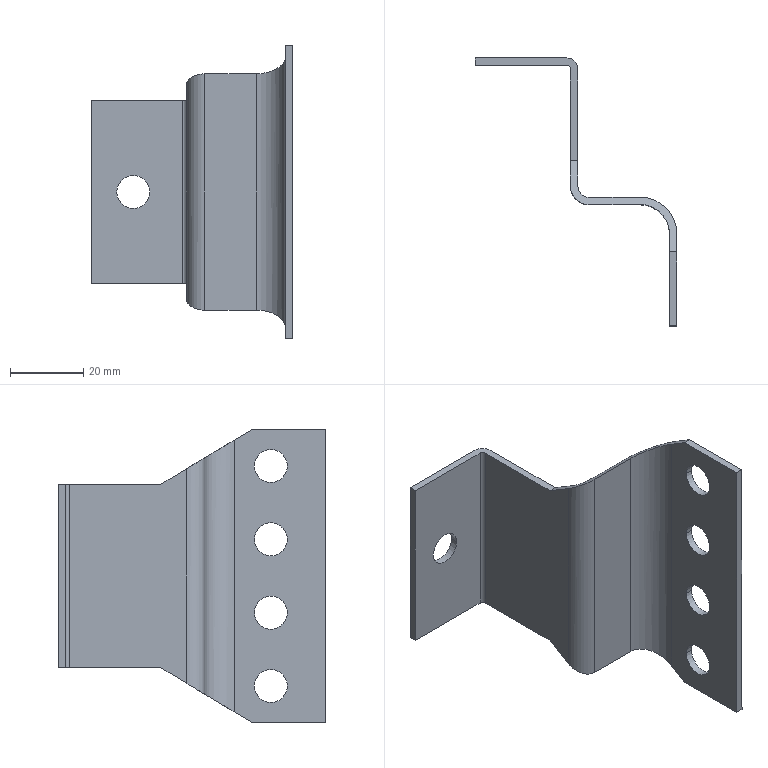Component | SolidWorks | 500CabinetWidthDoorCrossbeamAssembly-1_Connector-1 | 1 solid | 32 faces | box 55 x 73 x 80 mm | volume 13851 mm3 | cylinder 16 | plane 16 | commonest cylinder face diameters 9 x10 6 x2 20 x1 16 x1 10 x1 2 x1 | material Plain Carbon Steel
STEP:
#1=COLOUR_RGB('',0.7922,0.8196,0.9333);
#2=FILL_AREA_STYLE_COLOUR('',#1);
#3=FILL_AREA_STYLE('',(#2));
#4=SURFACE_STYLE_FILL_AREA(#3);
#5=SURFACE_SIDE_STYLE('',(#4));
#6=SURFACE_STYLE_USAGE(.BOTH.,#5);
#7=PRESENTATION_STYLE_ASSIGNMENT((#6));
#8=CARTESIAN_POINT('',(-49.801,4.761,85.05));
#9=VERTEX_POINT('',#8);
#10=CARTESIAN_POINT('',(-49.801,4.406,85.05));
#11=VERTEX_POINT('',#10);
#12=CARTESIAN_POINT('',(-49.801,4.583,85.05));
#13=DIRECTION('',(1.,0.,0.));
#14=DIRECTION('',(0.,-1.,0.));
#15=AXIS2_PLACEMENT_3D('',#12,#13,#14);
#16=CIRCLE('',#15,0.1772);
#17=EDGE_CURVE('',#9,#11,#16,.T.);
#18=ORIENTED_EDGE('',*,*,#17,.F.);
#19=CARTESIAN_POINT('',(-49.722,4.761,85.05));
#20=VERTEX_POINT('',#19);
#21=CARTESIAN_POINT('',(-52.872,4.761,85.05));
#22=DIRECTION('',(1.,-0.,0.));
#23=VECTOR('',#22,39.37);
#24=LINE('',#21,#23);
#25=EDGE_CURVE('',#9,#20,#24,.T.);
#26=ORIENTED_EDGE('',*,*,#25,.T.);
#27=CARTESIAN_POINT('',(-49.722,4.406,85.05));
#28=VERTEX_POINT('',#27);
#29=CARTESIAN_POINT('',(-49.722,4.583,85.05));
#30=DIRECTION('',(1.,-0.,0.));
#31=DIRECTION('',(0.,-1.,0.));
#32=AXIS2_PLACEMENT_3D('',#29,#30,#31);
#33=CIRCLE('',#32,0.1772);
#34=EDGE_CURVE('',#20,#28,#33,.T.);
#35=ORIENTED_EDGE('',*,*,#34,.T.);
#36=CARTESIAN_POINT('',(-52.872,4.406,85.05));
#37=DIRECTION('',(1.,-0.,0.));
#38=VECTOR('',#37,39.37);
#39=LINE('',#36,#38);
#40=EDGE_CURVE('',#11,#28,#39,.T.);
#41=ORIENTED_EDGE('',*,*,#40,.F.);
#42=EDGE_LOOP('',(#18,#26,#35,#41));
#43=FACE_OUTER_BOUND('',#42,.T.);
#44=CARTESIAN_POINT('',(-52.872,4.583,85.05));
#45=DIRECTION('',(1.,-0.,0.));
#46=DIRECTION('',(0.,-1.,0.));
#47=AXIS2_PLACEMENT_3D('',#44,#45,#46);
#48=CYLINDRICAL_SURFACE('',#47,0.1772);
#49=ADVANCED_FACE('',(#43),#48,.F.);
#50=CARTESIAN_POINT('',(-49.801,4.761,87.412));
#51=VERTEX_POINT('',#50);
#52=CARTESIAN_POINT('',(-49.801,4.406,87.412));
#53=VERTEX_POINT('',#52);
#54=CARTESIAN_POINT('',(-49.801,4.583,87.412));
#55=DIRECTION('',(1.,0.,0.));
#56=DIRECTION('',(0.,-1.,0.));
#57=AXIS2_PLACEMENT_3D('',#54,#55,#56);
#58=CIRCLE('',#57,0.1772);
#59=EDGE_CURVE('',#51,#53,#58,.T.);
#60=ORIENTED_EDGE('',*,*,#59,.F.);
#61=CARTESIAN_POINT('',(-49.722,4.761,87.412));
#62=VERTEX_POINT('',#61);
#63=CARTESIAN_POINT('',(-52.872,4.761,87.412));
#64=DIRECTION('',(1.,-0.,0.));
#65=VECTOR('',#64,39.37);
#66=LINE('',#63,#65);
#67=EDGE_CURVE('',#51,#62,#66,.T.);
#68=ORIENTED_EDGE('',*,*,#67,.T.);
#69=CARTESIAN_POINT('',(-49.722,4.406,87.412));
#70=VERTEX_POINT('',#69);
#71=CARTESIAN_POINT('',(-49.722,4.583,87.412));
#72=DIRECTION('',(1.,-0.,0.));
#73=DIRECTION('',(0.,-1.,0.));
#74=AXIS2_PLACEMENT_3D('',#71,#72,#73);
#75=CIRCLE('',#74,0.1772);
#76=EDGE_CURVE('',#62,#70,#75,.T.);
#77=ORIENTED_EDGE('',*,*,#76,.T.);
#78=CARTESIAN_POINT('',(-52.872,4.406,87.412));
#79=DIRECTION('',(1.,-0.,0.));
#80=VECTOR('',#79,39.37);
#81=LINE('',#78,#80);
#82=EDGE_CURVE('',#53,#70,#81,.T.);
#83=ORIENTED_EDGE('',*,*,#82,.F.);
#84=EDGE_LOOP('',(#60,#68,#77,#83));
#85=FACE_OUTER_BOUND('',#84,.T.);
#86=CARTESIAN_POINT('',(-52.872,4.583,87.412));
#87=DIRECTION('',(1.,-0.,0.));
#88=DIRECTION('',(0.,-1.,0.));
#89=AXIS2_PLACEMENT_3D('',#86,#87,#88);
#90=CYLINDRICAL_SURFACE('',#89,0.1772);
#91=ADVANCED_FACE('',(#85),#90,.F.);
#92=CARTESIAN_POINT('',(-49.801,4.761,86.625));
#93=VERTEX_POINT('',#92);
#94=CARTESIAN_POINT('',(-49.801,4.406,86.625));
#95=VERTEX_POINT('',#94);
#96=CARTESIAN_POINT('',(-49.801,4.583,86.625));
#97=DIRECTION('',(1.,0.,0.));
#98=DIRECTION('',(0.,-1.,0.));
#99=AXIS2_PLACEMENT_3D('',#96,#97,#98);
#100=CIRCLE('',#99,0.1772);
#101=EDGE_CURVE('',#93,#95,#100,.T.);
#102=ORIENTED_EDGE('',*,*,#101,.F.);
#103=CARTESIAN_POINT('',(-49.722,4.761,86.625));
#104=VERTEX_POINT('',#103);
#105=CARTESIAN_POINT('',(-52.872,4.761,86.625));
#106=DIRECTION('',(1.,-0.,0.));
#107=VECTOR('',#106,39.37);
#108=LINE('',#105,#107);
#109=EDGE_CURVE('',#93,#104,#108,.T.);
#110=ORIENTED_EDGE('',*,*,#109,.T.);
#111=CARTESIAN_POINT('',(-49.722,4.406,86.625));
#112=VERTEX_POINT('',#111);
#113=CARTESIAN_POINT('',(-49.722,4.583,86.625));
#114=DIRECTION('',(1.,-0.,0.));
#115=DIRECTION('',(0.,-1.,0.));
#116=AXIS2_PLACEMENT_3D('',#113,#114,#115);
#117=CIRCLE('',#116,0.1772);
#118=EDGE_CURVE('',#104,#112,#117,.T.);
#119=ORIENTED_EDGE('',*,*,#118,.T.);
#120=CARTESIAN_POINT('',(-52.872,4.406,86.625));
#121=DIRECTION('',(1.,-0.,0.));
#122=VECTOR('',#121,39.37);
#123=LINE('',#120,#122);
#124=EDGE_CURVE('',#95,#112,#123,.T.);
#125=ORIENTED_EDGE('',*,*,#124,.F.);
#126=EDGE_LOOP('',(#102,#110,#119,#125));
#127=FACE_OUTER_BOUND('',#126,.T.);
#128=CARTESIAN_POINT('',(-52.872,4.583,86.625));
#129=DIRECTION('',(1.,-0.,0.));
#130=DIRECTION('',(0.,-1.,0.));
#131=AXIS2_PLACEMENT_3D('',#128,#129,#130);
#132=CYLINDRICAL_SURFACE('',#131,0.1772);
#133=ADVANCED_FACE('',(#127),#132,.F.);
#134=CARTESIAN_POINT('',(-49.801,4.761,85.837));
#135=VERTEX_POINT('',#134);
#136=CARTESIAN_POINT('',(-49.801,4.406,85.837));
#137=VERTEX_POINT('',#136);
#138=CARTESIAN_POINT('',(-49.801,4.583,85.837));
#139=DIRECTION('',(1.,0.,0.));
#140=DIRECTION('',(0.,-1.,0.));
#141=AXIS2_PLACEMENT_3D('',#138,#139,#140);
#142=CIRCLE('',#141,0.1772);
#143=EDGE_CURVE('',#135,#137,#142,.T.);
#144=ORIENTED_EDGE('',*,*,#143,.F.);
#145=CARTESIAN_POINT('',(-49.722,4.761,85.837));
#146=VERTEX_POINT('',#145);
#147=CARTESIAN_POINT('',(-52.872,4.761,85.837));
#148=DIRECTION('',(1.,-0.,0.));
#149=VECTOR('',#148,39.37);
#150=LINE('',#147,#149);
#151=EDGE_CURVE('',#135,#146,#150,.T.);
#152=ORIENTED_EDGE('',*,*,#151,.T.);
#153=CARTESIAN_POINT('',(-49.722,4.406,85.837));
#154=VERTEX_POINT('',#153);
#155=CARTESIAN_POINT('',(-49.722,4.583,85.837));
#156=DIRECTION('',(1.,-0.,0.));
#157=DIRECTION('',(0.,-1.,0.));
#158=AXIS2_PLACEMENT_3D('',#155,#156,#157);
#159=CIRCLE('',#158,0.1772);
#160=EDGE_CURVE('',#146,#154,#159,.T.);
#161=ORIENTED_EDGE('',*,*,#160,.T.);
#162=CARTESIAN_POINT('',(-52.872,4.406,85.837));
#163=DIRECTION('',(1.,-0.,0.));
#164=VECTOR('',#163,39.37);
#165=LINE('',#162,#164);
#166=EDGE_CURVE('',#137,#154,#165,.T.);
#167=ORIENTED_EDGE('',*,*,#166,.F.);
#168=EDGE_LOOP('',(#144,#152,#161,#167));
#169=FACE_OUTER_BOUND('',#168,.T.);
#170=CARTESIAN_POINT('',(-52.872,4.583,85.837));
#171=DIRECTION('',(1.,-0.,0.));
#172=DIRECTION('',(0.,-1.,0.));
#173=AXIS2_PLACEMENT_3D('',#170,#171,#172);
#174=CYLINDRICAL_SURFACE('',#173,0.1772);
#175=ADVANCED_FACE('',(#169),#174,.F.);
#176=CARTESIAN_POINT('',(-51.612,6.788,86.231));
#177=VERTEX_POINT('',#176);
#178=CARTESIAN_POINT('',(-51.257,6.788,86.231));
#179=VERTEX_POINT('',#178);
#180=CARTESIAN_POINT('',(-51.435,6.788,86.231));
#181=DIRECTION('',(-0.,1.,-0.));
#182=DIRECTION('',(1.,0.,0.));
#183=AXIS2_PLACEMENT_3D('',#180,#181,#182);
#184=CIRCLE('',#183,0.1772);
#185=EDGE_CURVE('',#177,#179,#184,.T.);
#186=ORIENTED_EDGE('',*,*,#185,.F.);
#187=CARTESIAN_POINT('',(-51.612,6.867,86.231));
#188=VERTEX_POINT('',#187);
#189=CARTESIAN_POINT('',(-51.612,3.717,86.231));
#190=DIRECTION('',(-0.,1.,-0.));
#191=VECTOR('',#190,39.37);
#192=LINE('',#189,#191);
#193=EDGE_CURVE('',#177,#188,#192,.T.);
#194=ORIENTED_EDGE('',*,*,#193,.T.);
#195=CARTESIAN_POINT('',(-51.257,6.867,86.231));
#196=VERTEX_POINT('',#195);
#197=CARTESIAN_POINT('',(-51.435,6.867,86.231));
#198=DIRECTION('',(-0.,1.,-0.));
#199=DIRECTION('',(1.,0.,0.));
#200=AXIS2_PLACEMENT_3D('',#197,#198,#199);
#201=CIRCLE('',#200,0.1772);
#202=EDGE_CURVE('',#188,#196,#201,.T.);
#203=ORIENTED_EDGE('',*,*,#202,.T.);
#204=CARTESIAN_POINT('',(-51.257,3.717,86.231));
#205=DIRECTION('',(-0.,1.,-0.));
#206=VECTOR('',#205,39.37);
#207=LINE('',#204,#206);
#208=EDGE_CURVE('',#179,#196,#207,.T.);
#209=ORIENTED_EDGE('',*,*,#208,.F.);
#210=EDGE_LOOP('',(#186,#194,#203,#209));
#211=FACE_OUTER_BOUND('',#210,.T.);
#212=CARTESIAN_POINT('',(-51.435,3.717,86.231));
#213=DIRECTION('',(-0.,1.,-0.));
#214=DIRECTION('',(1.,0.,0.));
#215=AXIS2_PLACEMENT_3D('',#212,#213,#214);
#216=CYLINDRICAL_SURFACE('',#215,0.1772);
#217=ADVANCED_FACE('',(#211),#216,.F.);
#218=CARTESIAN_POINT('',(-51.435,6.788,86.231));
#219=DIRECTION('',(-0.,1.,-0.));
#220=DIRECTION('',(1.,0.,0.));
#221=AXIS2_PLACEMENT_3D('',#218,#219,#220);
#222=CIRCLE('',#221,0.1772);
#223=EDGE_CURVE('',#179,#177,#222,.T.);
#224=ORIENTED_EDGE('',*,*,#223,.T.);
#225=ORIENTED_EDGE('',*,*,#185,.T.);
#226=EDGE_LOOP('',(#224,#225));
#227=FACE_BOUND('',#226,.T.);
#228=CARTESIAN_POINT('',(-50.903,6.788,85.247));
#229=VERTEX_POINT('',#228);
#230=CARTESIAN_POINT('',(-51.887,6.788,85.247));
#231=VERTEX_POINT('',#230);
#232=CARTESIAN_POINT('',(-50.903,6.788,85.247));
#233=DIRECTION('',(-1.,-0.,-0.));
#234=VECTOR('',#233,39.37);
#235=LINE('',#232,#234);
#236=EDGE_CURVE('',#229,#231,#235,.T.);
#237=ORIENTED_EDGE('',*,*,#236,.F.);
#238=CARTESIAN_POINT('',(-50.903,6.788,87.215));
#239=VERTEX_POINT('',#238);
#240=CARTESIAN_POINT('',(-50.903,6.788,84.656));
#241=DIRECTION('',(-0.,0.,1.));
#242=VECTOR('',#241,39.37);
#243=LINE('',#240,#242);
#244=EDGE_CURVE('',#229,#239,#243,.T.);
#245=ORIENTED_EDGE('',*,*,#244,.T.);
#246=CARTESIAN_POINT('',(-51.887,6.788,87.215));
#247=VERTEX_POINT('',#246);
#248=CARTESIAN_POINT('',(-50.903,6.788,87.215));
#249=DIRECTION('',(1.,0.,0.));
#250=VECTOR('',#249,39.37);
#251=LINE('',#248,#250);
#252=EDGE_CURVE('',#247,#239,#251,.T.);
#253=ORIENTED_EDGE('',*,*,#252,.F.);
#254=CARTESIAN_POINT('',(-51.887,6.788,84.656));
#255=DIRECTION('',(-0.,0.,1.));
#256=VECTOR('',#255,39.37);
#257=LINE('',#254,#256);
#258=EDGE_CURVE('',#231,#247,#257,.T.);
#259=ORIENTED_EDGE('',*,*,#258,.F.);
#260=EDGE_LOOP('',(#237,#245,#253,#259));
#261=FACE_OUTER_BOUND('',#260,.T.);
#262=CARTESIAN_POINT('',(-50.903,6.788,84.656));
#263=DIRECTION('',(-0.,1.,-0.));
#264=DIRECTION('',(1.,0.,0.));
#265=AXIS2_PLACEMENT_3D('',#262,#263,#264);
#266=PLANE('',#265);
#267=ADVANCED_FACE('',(#227,#261),#266,.F.);
#268=CARTESIAN_POINT('',(-51.887,6.867,85.247));
#269=VERTEX_POINT('',#268);
#270=CARTESIAN_POINT('',(-51.887,6.867,87.215));
#271=VERTEX_POINT('',#270);
#272=CARTESIAN_POINT('',(-51.887,6.867,84.656));
#273=DIRECTION('',(-0.,0.,1.));
#274=VECTOR('',#273,39.37);
#275=LINE('',#272,#274);
#276=EDGE_CURVE('',#269,#271,#275,.T.);
#277=ORIENTED_EDGE('',*,*,#276,.F.);
#278=CARTESIAN_POINT('',(-51.887,5.764,85.247));
#279=DIRECTION('',(0.,-1.,0.));
#280=VECTOR('',#279,39.37);
#281=LINE('',#278,#280);
#282=EDGE_CURVE('',#269,#231,#281,.T.);
#283=ORIENTED_EDGE('',*,*,#282,.T.);
#284=ORIENTED_EDGE('',*,*,#258,.T.);
#285=CARTESIAN_POINT('',(-51.887,5.764,87.215));
#286=DIRECTION('',(-0.,1.,-0.));
#287=VECTOR('',#286,39.37);
#288=LINE('',#285,#287);
#289=EDGE_CURVE('',#247,#271,#288,.T.);
#290=ORIENTED_EDGE('',*,*,#289,.T.);
#291=EDGE_LOOP('',(#277,#283,#284,#290));
#292=FACE_OUTER_BOUND('',#291,.T.);
#293=CARTESIAN_POINT('',(-51.887,6.867,84.656));
#294=DIRECTION('',(-1.,-0.,-0.));
#295=DIRECTION('',(-0.,1.,-0.));
#296=AXIS2_PLACEMENT_3D('',#293,#294,#295);
#297=PLANE('',#296);
#298=ADVANCED_FACE('',(#292),#297,.T.);
#299=CARTESIAN_POINT('',(-51.435,6.867,86.231));
#300=DIRECTION('',(-0.,1.,-0.));
#301=DIRECTION('',(1.,0.,0.));
#302=AXIS2_PLACEMENT_3D('',#299,#300,#301);
#303=CIRCLE('',#302,0.1772);
#304=EDGE_CURVE('',#196,#188,#303,.T.);
#305=ORIENTED_EDGE('',*,*,#304,.F.);
#306=ORIENTED_EDGE('',*,*,#202,.F.);
#307=EDGE_LOOP('',(#305,#306));
#308=FACE_BOUND('',#307,.T.);
#309=CARTESIAN_POINT('',(-50.903,6.867,85.247));
#310=VERTEX_POINT('',#309);
#311=CARTESIAN_POINT('',(-50.903,6.867,87.215));
#312=VERTEX_POINT('',#311);
#313=CARTESIAN_POINT('',(-50.903,6.867,84.656));
#314=DIRECTION('',(-0.,0.,1.));
#315=VECTOR('',#314,39.37);
#316=LINE('',#313,#315);
#317=EDGE_CURVE('',#310,#312,#316,.T.);
#318=ORIENTED_EDGE('',*,*,#317,.F.);
#319=CARTESIAN_POINT('',(-48.738,6.867,85.247));
#320=DIRECTION('',(-1.,-0.,-0.));
#321=VECTOR('',#320,39.37);
#322=LINE('',#319,#321);
#323=EDGE_CURVE('',#310,#269,#322,.T.);
#324=ORIENTED_EDGE('',*,*,#323,.T.);
#325=ORIENTED_EDGE('',*,*,#276,.T.);
#326=CARTESIAN_POINT('',(-48.738,6.867,87.215));
#327=DIRECTION('',(-1.,-0.,-0.));
#328=VECTOR('',#327,39.37);
#329=LINE('',#326,#328);
#330=EDGE_CURVE('',#312,#271,#329,.T.);
#331=ORIENTED_EDGE('',*,*,#330,.F.);
#332=EDGE_LOOP('',(#318,#324,#325,#331));
#333=FACE_OUTER_BOUND('',#332,.T.);
#334=CARTESIAN_POINT('',(-50.903,6.867,84.656));
#335=DIRECTION('',(-0.,1.,-0.));
#336=DIRECTION('',(1.,0.,0.));
#337=AXIS2_PLACEMENT_3D('',#334,#335,#336);
#338=PLANE('',#337);
#339=ADVANCED_FACE('',(#308,#333),#338,.T.);
#340=CARTESIAN_POINT('',(-50.785,6.749,85.247));
#341=VERTEX_POINT('',#340);
#342=CARTESIAN_POINT('',(-50.785,6.749,87.215));
#343=VERTEX_POINT('',#342);
#344=CARTESIAN_POINT('',(-50.785,6.749,84.656));
#345=DIRECTION('',(-0.,0.,1.));
#346=VECTOR('',#345,39.37);
#347=LINE('',#344,#346);
#348=EDGE_CURVE('',#341,#343,#347,.T.);
#349=ORIENTED_EDGE('',*,*,#348,.F.);
#350=CARTESIAN_POINT('',(-50.903,6.749,85.247));
#351=DIRECTION('',(-0.,0.,1.));
#352=DIRECTION('',(-1.,0.,0.));
#353=AXIS2_PLACEMENT_3D('',#350,#351,#352);
#354=CIRCLE('',#353,0.1181);
#355=EDGE_CURVE('',#341,#310,#354,.T.);
#356=ORIENTED_EDGE('',*,*,#355,.T.);
#357=ORIENTED_EDGE('',*,*,#317,.T.);
#358=CARTESIAN_POINT('',(-50.903,6.749,87.215));
#359=DIRECTION('',(0.,-0.,-1.));
#360=DIRECTION('',(1.,0.,0.));
#361=AXIS2_PLACEMENT_3D('',#358,#359,#360);
#362=CIRCLE('',#361,0.1181);
#363=EDGE_CURVE('',#312,#343,#362,.T.);
#364=ORIENTED_EDGE('',*,*,#363,.T.);
#365=EDGE_LOOP('',(#349,#356,#357,#364));
#366=FACE_OUTER_BOUND('',#365,.T.);
#367=CARTESIAN_POINT('',(-50.903,6.749,84.656));
#368=DIRECTION('',(-0.,0.,1.));
#369=DIRECTION('',(1.,0.,0.));
#370=AXIS2_PLACEMENT_3D('',#367,#368,#369);
#371=CYLINDRICAL_SURFACE('',#370,0.1181);
#372=ADVANCED_FACE('',(#366),#371,.T.);
#373=CARTESIAN_POINT('',(-50.785,5.489,85.081));
#374=VERTEX_POINT('',#373);
#375=CARTESIAN_POINT('',(-50.785,5.489,87.381));
#376=VERTEX_POINT('',#375);
#377=CARTESIAN_POINT('',(-50.785,5.489,84.656));
#378=DIRECTION('',(-0.,0.,1.));
#379=VECTOR('',#378,39.37);
#380=LINE('',#377,#379);
#381=EDGE_CURVE('',#374,#376,#380,.T.);
#382=ORIENTED_EDGE('',*,*,#381,.F.);
#383=CARTESIAN_POINT('',(-50.785,5.764,85.247));
#384=VERTEX_POINT('',#383);
#385=CARTESIAN_POINT('',(-50.785,5.301,84.968));
#386=DIRECTION('',(-0.,0.8567,0.5157));
#387=VECTOR('',#386,39.37);
#388=LINE('',#385,#387);
#389=EDGE_CURVE('',#374,#384,#388,.T.);
#390=ORIENTED_EDGE('',*,*,#389,.T.);
#391=CARTESIAN_POINT('',(-50.785,5.489,85.247));
#392=DIRECTION('',(-0.,1.,-0.));
#393=VECTOR('',#392,39.37);
#394=LINE('',#391,#393);
#395=EDGE_CURVE('',#384,#341,#394,.T.);
#396=ORIENTED_EDGE('',*,*,#395,.T.);
#397=ORIENTED_EDGE('',*,*,#348,.T.);
#398=CARTESIAN_POINT('',(-50.785,5.764,87.215));
#399=VERTEX_POINT('',#398);
#400=CARTESIAN_POINT('',(-50.785,5.489,87.215));
#401=DIRECTION('',(0.,-1.,0.));
#402=VECTOR('',#401,39.37);
#403=LINE('',#400,#402);
#404=EDGE_CURVE('',#343,#399,#403,.T.);
#405=ORIENTED_EDGE('',*,*,#404,.T.);
#406=CARTESIAN_POINT('',(-50.785,6.693,86.656));
#407=DIRECTION('',(0.,-0.8567,0.5157));
#408=VECTOR('',#407,39.37);
#409=LINE('',#406,#408);
#410=EDGE_CURVE('',#399,#376,#409,.T.);
#411=ORIENTED_EDGE('',*,*,#410,.T.);
#412=EDGE_LOOP('',(#382,#390,#396,#397,#405,#411));
#413=FACE_OUTER_BOUND('',#412,.T.);
#414=CARTESIAN_POINT('',(-50.785,5.489,84.656));
#415=DIRECTION('',(1.,0.,0.));
#416=DIRECTION('',(0.,-1.,0.));
#417=AXIS2_PLACEMENT_3D('',#414,#415,#416);
#418=PLANE('',#417);
#419=ADVANCED_FACE('',(#413),#418,.T.);
#420=CARTESIAN_POINT('',(-50.667,5.371,85.01));
#421=VERTEX_POINT('',#420);
#422=CARTESIAN_POINT('',(-50.667,5.371,87.452));
#423=VERTEX_POINT('',#422);
#424=CARTESIAN_POINT('',(-50.667,5.371,84.656));
#425=DIRECTION('',(-0.,0.,1.));
#426=VECTOR('',#425,39.37);
#427=LINE('',#424,#426);
#428=EDGE_CURVE('',#421,#423,#427,.T.);
#429=ORIENTED_EDGE('',*,*,#428,.F.);
#430=CARTESIAN_POINT('',(-50.667,5.371,85.01));
#431=CARTESIAN_POINT('',(-50.736,5.371,85.01));
#432=CARTESIAN_POINT('',(-50.785,5.42,85.039));
#433=CARTESIAN_POINT('',(-50.785,5.489,85.081));
#434=(BOUNDED_CURVE()B_SPLINE_CURVE(3,(#430,#431,#432,#433),.UNSPECIFIED.,.F.,.F.)B_SPLINE_CURVE_WITH_KNOTS((4,4),(3.142,4.712),.UNSPECIFIED.)CURVE()GEOMETRIC_REPRESENTATION_ITEM()RATIONAL_B_SPLINE_CURVE((1.,0.8047,0.8047,1.))REPRESENTATION_ITEM(''));
#435=EDGE_CURVE('',#421,#374,#434,.T.);
#436=ORIENTED_EDGE('',*,*,#435,.T.);
#437=ORIENTED_EDGE('',*,*,#381,.T.);
#438=CARTESIAN_POINT('',(-50.785,5.489,87.381));
#439=CARTESIAN_POINT('',(-50.785,5.42,87.423));
#440=CARTESIAN_POINT('',(-50.736,5.371,87.452));
#441=CARTESIAN_POINT('',(-50.667,5.371,87.452));
#442=(BOUNDED_CURVE()B_SPLINE_CURVE(3,(#438,#439,#440,#441),.UNSPECIFIED.,.F.,.F.)B_SPLINE_CURVE_WITH_KNOTS((4,4),(4.712,6.283),.UNSPECIFIED.)CURVE()GEOMETRIC_REPRESENTATION_ITEM()RATIONAL_B_SPLINE_CURVE((1.,0.8047,0.8047,1.))REPRESENTATION_ITEM(''));
#443=EDGE_CURVE('',#376,#423,#442,.T.);
#444=ORIENTED_EDGE('',*,*,#443,.T.);
#445=EDGE_LOOP('',(#429,#436,#437,#444));
#446=FACE_OUTER_BOUND('',#445,.T.);
#447=CARTESIAN_POINT('',(-50.667,5.489,84.656));
#448=DIRECTION('',(-0.,0.,1.));
#449=DIRECTION('',(1.,0.,0.));
#450=AXIS2_PLACEMENT_3D('',#447,#448,#449);
#451=CYLINDRICAL_SURFACE('',#450,0.1181);
#452=ADVANCED_FACE('',(#446),#451,.F.);
#453=CARTESIAN_POINT('',(-50.116,5.371,85.01));
#454=VERTEX_POINT('',#453);
#455=CARTESIAN_POINT('',(-50.116,5.371,87.452));
#456=VERTEX_POINT('',#455);
#457=CARTESIAN_POINT('',(-50.116,5.371,84.656));
#458=DIRECTION('',(-0.,0.,1.));
#459=VECTOR('',#458,39.37);
#460=LINE('',#457,#459);
#461=EDGE_CURVE('',#454,#456,#460,.T.);
#462=ORIENTED_EDGE('',*,*,#461,.F.);
#463=CARTESIAN_POINT('',(-50.116,5.371,85.01));
#464=DIRECTION('',(-1.,-0.,-0.));
#465=VECTOR('',#464,39.37);
#466=LINE('',#463,#465);
#467=EDGE_CURVE('',#454,#421,#466,.T.);
#468=ORIENTED_EDGE('',*,*,#467,.T.);
#469=ORIENTED_EDGE('',*,*,#428,.T.);
#470=CARTESIAN_POINT('',(-50.116,5.371,87.452));
#471=DIRECTION('',(1.,0.,0.));
#472=VECTOR('',#471,39.37);
#473=LINE('',#470,#472);
#474=EDGE_CURVE('',#423,#456,#473,.T.);
#475=ORIENTED_EDGE('',*,*,#474,.T.);
#476=EDGE_LOOP('',(#462,#468,#469,#475));
#477=FACE_OUTER_BOUND('',#476,.T.);
#478=CARTESIAN_POINT('',(-50.116,5.371,84.656));
#479=DIRECTION('',(-0.,1.,-0.));
#480=DIRECTION('',(1.,0.,0.));
#481=AXIS2_PLACEMENT_3D('',#478,#479,#480);
#482=PLANE('',#481);
#483=ADVANCED_FACE('',(#477),#482,.T.);
#484=CARTESIAN_POINT('',(-49.722,4.977,84.773));
#485=VERTEX_POINT('',#484);
#486=CARTESIAN_POINT('',(-49.722,4.977,87.689));
#487=VERTEX_POINT('',#486);
#488=CARTESIAN_POINT('',(-49.722,4.977,84.656));
#489=DIRECTION('',(-0.,0.,1.));
#490=VECTOR('',#489,39.37);
#491=LINE('',#488,#490);
#492=EDGE_CURVE('',#485,#487,#491,.T.);
#493=ORIENTED_EDGE('',*,*,#492,.F.);
#494=CARTESIAN_POINT('',(-49.722,4.977,84.773));
#495=CARTESIAN_POINT('',(-49.722,5.208,84.912));
#496=CARTESIAN_POINT('',(-49.885,5.371,85.01));
#497=CARTESIAN_POINT('',(-50.116,5.371,85.01));
#498=(BOUNDED_CURVE()B_SPLINE_CURVE(3,(#494,#495,#496,#497),.UNSPECIFIED.,.F.,.F.)B_SPLINE_CURVE_WITH_KNOTS((4,4),(4.712,6.283),.UNSPECIFIED.)CURVE()GEOMETRIC_REPRESENTATION_ITEM()RATIONAL_B_SPLINE_CURVE((1.,0.8047,0.8047,1.))REPRESENTATION_ITEM(''));
#499=EDGE_CURVE('',#485,#454,#498,.T.);
#500=ORIENTED_EDGE('',*,*,#499,.T.);
#501=ORIENTED_EDGE('',*,*,#461,.T.);
#502=CARTESIAN_POINT('',(-50.116,5.371,87.452));
#503=CARTESIAN_POINT('',(-49.885,5.371,87.452));
#504=CARTESIAN_POINT('',(-49.722,5.208,87.551));
#505=CARTESIAN_POINT('',(-49.722,4.977,87.689));
#506=(BOUNDED_CURVE()B_SPLINE_CURVE(3,(#502,#503,#504,#505),.UNSPECIFIED.,.F.,.F.)B_SPLINE_CURVE_WITH_KNOTS((4,4),(3.142,4.712),.UNSPECIFIED.)CURVE()GEOMETRIC_REPRESENTATION_ITEM()RATIONAL_B_SPLINE_CURVE((1.,0.8047,0.8047,1.))REPRESENTATION_ITEM(''));
#507=EDGE_CURVE('',#456,#487,#506,.T.);
#508=ORIENTED_EDGE('',*,*,#507,.T.);
#509=EDGE_LOOP('',(#493,#500,#501,#508));
#510=FACE_OUTER_BOUND('',#509,.T.);
#511=CARTESIAN_POINT('',(-50.116,4.977,84.656));
#512=DIRECTION('',(-0.,0.,1.));
#513=DIRECTION('',(1.,0.,0.));
#514=AXIS2_PLACEMENT_3D('',#511,#512,#513);
#515=CYLINDRICAL_SURFACE('',#514,0.3937);
#516=ADVANCED_FACE('',(#510),#515,.T.);
#517=CARTESIAN_POINT('',(-49.722,4.583,85.05));
#518=DIRECTION('',(1.,-0.,0.));
#519=DIRECTION('',(0.,-1.,0.));
#520=AXIS2_PLACEMENT_3D('',#517,#518,#519);
#521=CIRCLE('',#520,0.1772);
#522=EDGE_CURVE('',#28,#20,#521,.T.);
#523=ORIENTED_EDGE('',*,*,#522,.F.);
#524=ORIENTED_EDGE('',*,*,#34,.F.);
#525=EDGE_LOOP('',(#523,#524));
#526=FACE_BOUND('',#525,.T.);
#527=CARTESIAN_POINT('',(-49.722,4.583,87.412));
#528=DIRECTION('',(1.,-0.,0.));
#529=DIRECTION('',(0.,-1.,0.));
#530=AXIS2_PLACEMENT_3D('',#527,#528,#529);
#531=CIRCLE('',#530,0.1772);
#532=EDGE_CURVE('',#70,#62,#531,.T.);
#533=ORIENTED_EDGE('',*,*,#532,.F.);
#534=ORIENTED_EDGE('',*,*,#76,.F.);
#535=EDGE_LOOP('',(#533,#534));
#536=FACE_BOUND('',#535,.T.);
#537=CARTESIAN_POINT('',(-49.722,4.583,86.625));
#538=DIRECTION('',(1.,-0.,0.));
#539=DIRECTION('',(0.,-1.,0.));
#540=AXIS2_PLACEMENT_3D('',#537,#538,#539);
#541=CIRCLE('',#540,0.1772);
#542=EDGE_CURVE('',#112,#104,#541,.T.);
#543=ORIENTED_EDGE('',*,*,#542,.F.);
#544=ORIENTED_EDGE('',*,*,#118,.F.);
#545=EDGE_LOOP('',(#543,#544));
#546=FACE_BOUND('',#545,.T.);
#547=CARTESIAN_POINT('',(-49.722,4.583,85.837));
#548=DIRECTION('',(1.,-0.,0.));
#549=DIRECTION('',(0.,-1.,0.));
#550=AXIS2_PLACEMENT_3D('',#547,#548,#549);
#551=CIRCLE('',#550,0.1772);
#552=EDGE_CURVE('',#154,#146,#551,.T.);
#553=ORIENTED_EDGE('',*,*,#552,.F.);
#554=ORIENTED_EDGE('',*,*,#160,.F.);
#555=EDGE_LOOP('',(#553,#554));
#556=FACE_BOUND('',#555,.T.);
#557=CARTESIAN_POINT('',(-49.722,3.993,84.656));
#558=VERTEX_POINT('',#557);
#559=CARTESIAN_POINT('',(-49.722,4.783,84.656));
#560=VERTEX_POINT('',#559);
#561=CARTESIAN_POINT('',(-49.722,3.993,84.656));
#562=DIRECTION('',(-0.,1.,-0.));
#563=VECTOR('',#562,39.37);
#564=LINE('',#561,#563);
#565=EDGE_CURVE('',#558,#560,#564,.T.);
#566=ORIENTED_EDGE('',*,*,#565,.T.);
#567=CARTESIAN_POINT('',(-49.722,4.203,84.307));
#568=DIRECTION('',(-0.,0.8567,0.5157));
#569=VECTOR('',#568,39.37);
#570=LINE('',#567,#569);
#571=EDGE_CURVE('',#560,#485,#570,.T.);
#572=ORIENTED_EDGE('',*,*,#571,.T.);
#573=ORIENTED_EDGE('',*,*,#492,.T.);
#574=CARTESIAN_POINT('',(-49.722,4.783,87.806));
#575=VERTEX_POINT('',#574);
#576=CARTESIAN_POINT('',(-49.722,5.595,87.317));
#577=DIRECTION('',(0.,-0.8567,0.5157));
#578=VECTOR('',#577,39.37);
#579=LINE('',#576,#578);
#580=EDGE_CURVE('',#487,#575,#579,.T.);
#581=ORIENTED_EDGE('',*,*,#580,.T.);
#582=CARTESIAN_POINT('',(-49.722,3.993,87.806));
#583=VERTEX_POINT('',#582);
#584=CARTESIAN_POINT('',(-49.722,3.993,87.806));
#585=DIRECTION('',(-0.,1.,-0.));
#586=VECTOR('',#585,39.37);
#587=LINE('',#584,#586);
#588=EDGE_CURVE('',#583,#575,#587,.T.);
#589=ORIENTED_EDGE('',*,*,#588,.F.);
#590=CARTESIAN_POINT('',(-49.722,3.993,84.656));
#591=DIRECTION('',(-0.,0.,1.));
#592=VECTOR('',#591,39.37);
#593=LINE('',#590,#592);
#594=EDGE_CURVE('',#558,#583,#593,.T.);
#595=ORIENTED_EDGE('',*,*,#594,.F.);
#596=EDGE_LOOP('',(#566,#572,#573,#581,#589,#595));
#597=FACE_OUTER_BOUND('',#596,.T.);
#598=CARTESIAN_POINT('',(-49.722,3.993,84.656));
#599=DIRECTION('',(1.,0.,0.));
#600=DIRECTION('',(0.,-1.,0.));
#601=AXIS2_PLACEMENT_3D('',#598,#599,#600);
#602=PLANE('',#601);
#603=ADVANCED_FACE('',(#526,#536,#546,#556,#597),#602,.T.);
#604=CARTESIAN_POINT('',(-49.801,4.583,85.05));
#605=DIRECTION('',(1.,0.,0.));
#606=DIRECTION('',(0.,-1.,0.));
#607=AXIS2_PLACEMENT_3D('',#604,#605,#606);
#608=CIRCLE('',#607,0.1772);
#609=EDGE_CURVE('',#11,#9,#608,.T.);
#610=ORIENTED_EDGE('',*,*,#609,.T.);
#611=ORIENTED_EDGE('',*,*,#17,.T.);
#612=EDGE_LOOP('',(#610,#611));
#613=FACE_BOUND('',#612,.T.);
#614=CARTESIAN_POINT('',(-49.801,4.583,87.412));
#615=DIRECTION('',(1.,0.,0.));
#616=DIRECTION('',(0.,-1.,0.));
#617=AXIS2_PLACEMENT_3D('',#614,#615,#616);
#618=CIRCLE('',#617,0.1772);
#619=EDGE_CURVE('',#53,#51,#618,.T.);
#620=ORIENTED_EDGE('',*,*,#619,.T.);
#621=ORIENTED_EDGE('',*,*,#59,.T.);
#622=EDGE_LOOP('',(#620,#621));
#623=FACE_BOUND('',#622,.T.);
#624=CARTESIAN_POINT('',(-49.801,4.583,86.625));
#625=DIRECTION('',(1.,0.,0.));
#626=DIRECTION('',(0.,-1.,0.));
#627=AXIS2_PLACEMENT_3D('',#624,#625,#626);
#628=CIRCLE('',#627,0.1772);
#629=EDGE_CURVE('',#95,#93,#628,.T.);
#630=ORIENTED_EDGE('',*,*,#629,.T.);
#631=ORIENTED_EDGE('',*,*,#101,.T.);
#632=EDGE_LOOP('',(#630,#631));
#633=FACE_BOUND('',#632,.T.);
#634=CARTESIAN_POINT('',(-49.801,4.583,85.837));
#635=DIRECTION('',(1.,0.,0.));
#636=DIRECTION('',(0.,-1.,0.));
#637=AXIS2_PLACEMENT_3D('',#634,#635,#636);
#638=CIRCLE('',#637,0.1772);
#639=EDGE_CURVE('',#137,#135,#638,.T.);
#640=ORIENTED_EDGE('',*,*,#639,.T.);
#641=ORIENTED_EDGE('',*,*,#143,.T.);
#642=EDGE_LOOP('',(#640,#641));
#643=FACE_BOUND('',#642,.T.);
#644=CARTESIAN_POINT('',(-49.801,4.783,84.656));
#645=VERTEX_POINT('',#644);
#646=CARTESIAN_POINT('',(-49.801,4.977,84.773));
#647=VERTEX_POINT('',#646);
#648=CARTESIAN_POINT('',(-49.801,4.203,84.307));
#649=DIRECTION('',(-0.,0.8567,0.5157));
#650=VECTOR('',#649,39.37);
#651=LINE('',#648,#650);
#652=EDGE_CURVE('',#645,#647,#651,.T.);
#653=ORIENTED_EDGE('',*,*,#652,.F.);
#654=CARTESIAN_POINT('',(-49.801,3.993,84.656));
#655=VERTEX_POINT('',#654);
#656=CARTESIAN_POINT('',(-49.801,3.993,84.656));
#657=DIRECTION('',(-0.,1.,-0.));
#658=VECTOR('',#657,39.37);
#659=LINE('',#656,#658);
#660=EDGE_CURVE('',#655,#645,#659,.T.);
#661=ORIENTED_EDGE('',*,*,#660,.F.);
#662=CARTESIAN_POINT('',(-49.801,3.993,87.806));
#663=VERTEX_POINT('',#662);
#664=CARTESIAN_POINT('',(-49.801,3.993,84.656));
#665=DIRECTION('',(-0.,0.,1.));
#666=VECTOR('',#665,39.37);
#667=LINE('',#664,#666);
#668=EDGE_CURVE('',#655,#663,#667,.T.);
#669=ORIENTED_EDGE('',*,*,#668,.T.);
#670=CARTESIAN_POINT('',(-49.801,4.783,87.806));
#671=VERTEX_POINT('',#670);
#672=CARTESIAN_POINT('',(-49.801,3.993,87.806));
#673=DIRECTION('',(-0.,1.,-0.));
#674=VECTOR('',#673,39.37);
#675=LINE('',#672,#674);
#676=EDGE_CURVE('',#663,#671,#675,.T.);
#677=ORIENTED_EDGE('',*,*,#676,.T.);
#678=CARTESIAN_POINT('',(-49.801,4.977,87.689));
#679=VERTEX_POINT('',#678);
#680=CARTESIAN_POINT('',(-49.801,5.595,87.317));
#681=DIRECTION('',(0.,-0.8567,0.5157));
#682=VECTOR('',#681,39.37);
#683=LINE('',#680,#682);
#684=EDGE_CURVE('',#679,#671,#683,.T.);
#685=ORIENTED_EDGE('',*,*,#684,.F.);
#686=CARTESIAN_POINT('',(-49.801,4.977,84.656));
#687=DIRECTION('',(-0.,0.,1.));
#688=VECTOR('',#687,39.37);
#689=LINE('',#686,#688);
#690=EDGE_CURVE('',#647,#679,#689,.T.);
#691=ORIENTED_EDGE('',*,*,#690,.F.);
#692=EDGE_LOOP('',(#653,#661,#669,#677,#685,#691));
#693=FACE_OUTER_BOUND('',#692,.T.);
#694=CARTESIAN_POINT('',(-49.801,3.993,84.656));
#695=DIRECTION('',(1.,0.,0.));
#696=DIRECTION('',(0.,-1.,0.));
#697=AXIS2_PLACEMENT_3D('',#694,#695,#696);
#698=PLANE('',#697);
#699=ADVANCED_FACE('',(#613,#623,#633,#643,#693),#698,.F.);
#700=CARTESIAN_POINT('',(-50.116,5.292,84.962));
#701=VERTEX_POINT('',#700);
#702=CARTESIAN_POINT('',(-49.801,4.977,84.773));
#703=CARTESIAN_POINT('',(-49.801,5.162,84.884));
#704=CARTESIAN_POINT('',(-49.931,5.292,84.962));
#705=CARTESIAN_POINT('',(-50.116,5.292,84.962));
#706=(BOUNDED_CURVE()B_SPLINE_CURVE(3,(#702,#703,#704,#705),.UNSPECIFIED.,.F.,.F.)B_SPLINE_CURVE_WITH_KNOTS((4,4),(4.712,6.283),.UNSPECIFIED.)CURVE()GEOMETRIC_REPRESENTATION_ITEM()RATIONAL_B_SPLINE_CURVE((1.,0.8047,0.8047,1.))REPRESENTATION_ITEM(''));
#707=EDGE_CURVE('',#647,#701,#706,.T.);
#708=ORIENTED_EDGE('',*,*,#707,.F.);
#709=ORIENTED_EDGE('',*,*,#690,.T.);
#710=CARTESIAN_POINT('',(-50.116,5.292,87.5));
#711=VERTEX_POINT('',#710);
#712=CARTESIAN_POINT('',(-50.116,5.292,87.5));
#713=CARTESIAN_POINT('',(-49.931,5.292,87.5));
#714=CARTESIAN_POINT('',(-49.801,5.162,87.578));
#715=CARTESIAN_POINT('',(-49.801,4.977,87.689));
#716=(BOUNDED_CURVE()B_SPLINE_CURVE(3,(#712,#713,#714,#715),.UNSPECIFIED.,.F.,.F.)B_SPLINE_CURVE_WITH_KNOTS((4,4),(3.142,4.712),.UNSPECIFIED.)CURVE()GEOMETRIC_REPRESENTATION_ITEM()RATIONAL_B_SPLINE_CURVE((1.,0.8047,0.8047,1.))REPRESENTATION_ITEM(''));
#717=EDGE_CURVE('',#711,#679,#716,.T.);
#718=ORIENTED_EDGE('',*,*,#717,.F.);
#719=CARTESIAN_POINT('',(-50.116,5.292,84.656));
#720=DIRECTION('',(-0.,0.,1.));
#721=VECTOR('',#720,39.37);
#722=LINE('',#719,#721);
#723=EDGE_CURVE('',#701,#711,#722,.T.);
#724=ORIENTED_EDGE('',*,*,#723,.F.);
#725=EDGE_LOOP('',(#708,#709,#718,#724));
#726=FACE_OUTER_BOUND('',#725,.T.);
#727=CARTESIAN_POINT('',(-50.116,4.977,84.656));
#728=DIRECTION('',(-0.,0.,1.));
#729=DIRECTION('',(1.,0.,0.));
#730=AXIS2_PLACEMENT_3D('',#727,#728,#729);
#731=CYLINDRICAL_SURFACE('',#730,0.315);
#732=ADVANCED_FACE('',(#726),#731,.F.);
#733=CARTESIAN_POINT('',(-50.667,5.292,84.962));
#734=VERTEX_POINT('',#733);
#735=CARTESIAN_POINT('',(-50.116,5.292,84.962));
#736=DIRECTION('',(-1.,-0.,-0.));
#737=VECTOR('',#736,39.37);
#738=LINE('',#735,#737);
#739=EDGE_CURVE('',#701,#734,#738,.T.);
#740=ORIENTED_EDGE('',*,*,#739,.F.);
#741=ORIENTED_EDGE('',*,*,#723,.T.);
#742=CARTESIAN_POINT('',(-50.667,5.292,87.5));
#743=VERTEX_POINT('',#742);
#744=CARTESIAN_POINT('',(-50.116,5.292,87.5));
#745=DIRECTION('',(1.,0.,0.));
#746=VECTOR('',#745,39.37);
#747=LINE('',#744,#746);
#748=EDGE_CURVE('',#743,#711,#747,.T.);
#749=ORIENTED_EDGE('',*,*,#748,.F.);
#750=CARTESIAN_POINT('',(-50.667,5.292,84.656));
#751=DIRECTION('',(-0.,0.,1.));
#752=VECTOR('',#751,39.37);
#753=LINE('',#750,#752);
#754=EDGE_CURVE('',#734,#743,#753,.T.);
#755=ORIENTED_EDGE('',*,*,#754,.F.);
#756=EDGE_LOOP('',(#740,#741,#749,#755));
#757=FACE_OUTER_BOUND('',#756,.T.);
#758=CARTESIAN_POINT('',(-50.116,5.292,84.656));
#759=DIRECTION('',(-0.,1.,-0.));
#760=DIRECTION('',(1.,0.,0.));
#761=AXIS2_PLACEMENT_3D('',#758,#759,#760);
#762=PLANE('',#761);
#763=ADVANCED_FACE('',(#757),#762,.F.);
#764=CARTESIAN_POINT('',(-50.864,5.489,85.081));
#765=VERTEX_POINT('',#764);
#766=CARTESIAN_POINT('',(-50.667,5.292,84.962));
#767=CARTESIAN_POINT('',(-50.782,5.292,84.962));
#768=CARTESIAN_POINT('',(-50.864,5.374,85.012));
#769=CARTESIAN_POINT('',(-50.864,5.489,85.081));
#770=(BOUNDED_CURVE()B_SPLINE_CURVE(3,(#766,#767,#768,#769),.UNSPECIFIED.,.F.,.F.)B_SPLINE_CURVE_WITH_KNOTS((4,4),(3.142,4.712),.UNSPECIFIED.)CURVE()GEOMETRIC_REPRESENTATION_ITEM()RATIONAL_B_SPLINE_CURVE((1.,0.8047,0.8047,1.))REPRESENTATION_ITEM(''));
#771=EDGE_CURVE('',#734,#765,#770,.T.);
#772=ORIENTED_EDGE('',*,*,#771,.F.);
#773=ORIENTED_EDGE('',*,*,#754,.T.);
#774=CARTESIAN_POINT('',(-50.864,5.489,87.381));
#775=VERTEX_POINT('',#774);
#776=CARTESIAN_POINT('',(-50.864,5.489,87.381));
#777=CARTESIAN_POINT('',(-50.864,5.374,87.451));
#778=CARTESIAN_POINT('',(-50.782,5.292,87.5));
#779=CARTESIAN_POINT('',(-50.667,5.292,87.5));
#780=(BOUNDED_CURVE()B_SPLINE_CURVE(3,(#776,#777,#778,#779),.UNSPECIFIED.,.F.,.F.)B_SPLINE_CURVE_WITH_KNOTS((4,4),(4.712,6.283),.UNSPECIFIED.)CURVE()GEOMETRIC_REPRESENTATION_ITEM()RATIONAL_B_SPLINE_CURVE((1.,0.8047,0.8047,1.))REPRESENTATION_ITEM(''));
#781=EDGE_CURVE('',#775,#743,#780,.T.);
#782=ORIENTED_EDGE('',*,*,#781,.F.);
#783=CARTESIAN_POINT('',(-50.864,5.489,84.656));
#784=DIRECTION('',(-0.,0.,1.));
#785=VECTOR('',#784,39.37);
#786=LINE('',#783,#785);
#787=EDGE_CURVE('',#765,#775,#786,.T.);
#788=ORIENTED_EDGE('',*,*,#787,.F.);
#789=EDGE_LOOP('',(#772,#773,#782,#788));
#790=FACE_OUTER_BOUND('',#789,.T.);
#791=CARTESIAN_POINT('',(-50.667,5.489,84.656));
#792=DIRECTION('',(-0.,0.,1.));
#793=DIRECTION('',(1.,0.,0.));
#794=AXIS2_PLACEMENT_3D('',#791,#792,#793);
#795=CYLINDRICAL_SURFACE('',#794,0.1969);
#796=ADVANCED_FACE('',(#790),#795,.T.);
#797=CARTESIAN_POINT('',(-50.864,5.764,85.247));
#798=VERTEX_POINT('',#797);
#799=CARTESIAN_POINT('',(-50.864,5.301,84.968));
#800=DIRECTION('',(-0.,0.8567,0.5157));
#801=VECTOR('',#800,39.37);
#802=LINE('',#799,#801);
#803=EDGE_CURVE('',#765,#798,#802,.T.);
#804=ORIENTED_EDGE('',*,*,#803,.F.);
#805=ORIENTED_EDGE('',*,*,#787,.T.);
#806=CARTESIAN_POINT('',(-50.864,5.764,87.215));
#807=VERTEX_POINT('',#806);
#808=CARTESIAN_POINT('',(-50.864,6.693,86.656));
#809=DIRECTION('',(0.,-0.8567,0.5157));
#810=VECTOR('',#809,39.37);
#811=LINE('',#808,#810);
#812=EDGE_CURVE('',#807,#775,#811,.T.);
#813=ORIENTED_EDGE('',*,*,#812,.F.);
#814=CARTESIAN_POINT('',(-50.864,6.749,87.215));
#815=VERTEX_POINT('',#814);
#816=CARTESIAN_POINT('',(-50.864,5.489,87.215));
#817=DIRECTION('',(0.,-1.,0.));
#818=VECTOR('',#817,39.37);
#819=LINE('',#816,#818);
#820=EDGE_CURVE('',#815,#807,#819,.T.);
#821=ORIENTED_EDGE('',*,*,#820,.F.);
#822=CARTESIAN_POINT('',(-50.864,6.749,85.247));
#823=VERTEX_POINT('',#822);
#824=CARTESIAN_POINT('',(-50.864,6.749,84.656));
#825=DIRECTION('',(-0.,0.,1.));
#826=VECTOR('',#825,39.37);
#827=LINE('',#824,#826);
#828=EDGE_CURVE('',#823,#815,#827,.T.);
#829=ORIENTED_EDGE('',*,*,#828,.F.);
#830=CARTESIAN_POINT('',(-50.864,5.489,85.247));
#831=DIRECTION('',(-0.,1.,-0.));
#832=VECTOR('',#831,39.37);
#833=LINE('',#830,#832);
#834=EDGE_CURVE('',#798,#823,#833,.T.);
#835=ORIENTED_EDGE('',*,*,#834,.F.);
#836=EDGE_LOOP('',(#804,#805,#813,#821,#829,#835));
#837=FACE_OUTER_BOUND('',#836,.T.);
#838=CARTESIAN_POINT('',(-50.864,5.489,84.656));
#839=DIRECTION('',(1.,0.,0.));
#840=DIRECTION('',(0.,-1.,0.));
#841=AXIS2_PLACEMENT_3D('',#838,#839,#840);
#842=PLANE('',#841);
#843=ADVANCED_FACE('',(#837),#842,.F.);
#844=CARTESIAN_POINT('',(-50.903,6.749,85.247));
#845=DIRECTION('',(-0.,0.,1.));
#846=DIRECTION('',(-1.,0.,0.));
#847=AXIS2_PLACEMENT_3D('',#844,#845,#846);
#848=CIRCLE('',#847,0.03937);
#849=EDGE_CURVE('',#823,#229,#848,.T.);
#850=ORIENTED_EDGE('',*,*,#849,.F.);
#851=ORIENTED_EDGE('',*,*,#828,.T.);
#852=CARTESIAN_POINT('',(-50.903,6.749,87.215));
#853=DIRECTION('',(0.,-0.,-1.));
#854=DIRECTION('',(1.,0.,0.));
#855=AXIS2_PLACEMENT_3D('',#852,#853,#854);
#856=CIRCLE('',#855,0.03937);
#857=EDGE_CURVE('',#239,#815,#856,.T.);
#858=ORIENTED_EDGE('',*,*,#857,.F.);
#859=ORIENTED_EDGE('',*,*,#244,.F.);
#860=EDGE_LOOP('',(#850,#851,#858,#859));
#861=FACE_OUTER_BOUND('',#860,.T.);
#862=CARTESIAN_POINT('',(-50.903,6.749,84.656));
#863=DIRECTION('',(-0.,0.,1.));
#864=DIRECTION('',(1.,0.,0.));
#865=AXIS2_PLACEMENT_3D('',#862,#863,#864);
#866=CYLINDRICAL_SURFACE('',#865,0.03937);
#867=ADVANCED_FACE('',(#861),#866,.F.);
#868=CARTESIAN_POINT('',(-50.903,4.783,84.656));
#869=DIRECTION('',(-1.,-0.,-0.));
#870=VECTOR('',#869,39.37);
#871=LINE('',#868,#870);
#872=EDGE_CURVE('',#560,#645,#871,.T.);
#873=ORIENTED_EDGE('',*,*,#872,.F.);
#874=ORIENTED_EDGE('',*,*,#565,.F.);
#875=CARTESIAN_POINT('',(-49.801,3.993,84.656));
#876=DIRECTION('',(1.,0.,0.));
#877=VECTOR('',#876,39.37);
#878=LINE('',#875,#877);
#879=EDGE_CURVE('',#655,#558,#878,.T.);
#880=ORIENTED_EDGE('',*,*,#879,.F.);
#881=ORIENTED_EDGE('',*,*,#660,.T.);
#882=EDGE_LOOP('',(#873,#874,#880,#881));
#883=FACE_OUTER_BOUND('',#882,.T.);
#884=CARTESIAN_POINT('',(-50.903,6.749,84.656));
#885=DIRECTION('',(-0.,0.,1.));
#886=DIRECTION('',(1.,0.,0.));
#887=AXIS2_PLACEMENT_3D('',#884,#885,#886);
#888=PLANE('',#887);
#889=ADVANCED_FACE('',(#883),#888,.F.);
#890=ORIENTED_EDGE('',*,*,#588,.T.);
#891=CARTESIAN_POINT('',(-50.903,4.783,87.806));
#892=DIRECTION('',(-1.,-0.,-0.));
#893=VECTOR('',#892,39.37);
#894=LINE('',#891,#893);
#895=EDGE_CURVE('',#575,#671,#894,.T.);
#896=ORIENTED_EDGE('',*,*,#895,.T.);
#897=ORIENTED_EDGE('',*,*,#676,.F.);
#898=CARTESIAN_POINT('',(-49.801,3.993,87.806));
#899=DIRECTION('',(1.,0.,0.));
#900=VECTOR('',#899,39.37);
#901=LINE('',#898,#900);
#902=EDGE_CURVE('',#663,#583,#901,.T.);
#903=ORIENTED_EDGE('',*,*,#902,.T.);
#904=EDGE_LOOP('',(#890,#896,#897,#903));
#905=FACE_OUTER_BOUND('',#904,.T.);
#906=CARTESIAN_POINT('',(-50.903,6.749,87.806));
#907=DIRECTION('',(-0.,0.,1.));
#908=DIRECTION('',(1.,0.,0.));
#909=AXIS2_PLACEMENT_3D('',#906,#907,#908);
#910=PLANE('',#909);
#911=ADVANCED_FACE('',(#905),#910,.T.);
#912=ORIENTED_EDGE('',*,*,#902,.F.);
#913=ORIENTED_EDGE('',*,*,#668,.F.);
#914=ORIENTED_EDGE('',*,*,#879,.T.);
#915=ORIENTED_EDGE('',*,*,#594,.T.);
#916=EDGE_LOOP('',(#912,#913,#914,#915));
#917=FACE_OUTER_BOUND('',#916,.T.);
#918=CARTESIAN_POINT('',(-49.801,3.993,84.656));
#919=DIRECTION('',(0.,-1.,0.));
#920=DIRECTION('',(-1.,-0.,-0.));
#921=AXIS2_PLACEMENT_3D('',#918,#919,#920);
#922=PLANE('',#921);
#923=ADVANCED_FACE('',(#917),#922,.T.);
#924=CARTESIAN_POINT('',(-48.738,5.764,87.215));
#925=DIRECTION('',(-1.,-0.,-0.));
#926=VECTOR('',#925,39.37);
#927=LINE('',#924,#926);
#928=EDGE_CURVE('',#399,#807,#927,.T.);
#929=ORIENTED_EDGE('',*,*,#928,.T.);
#930=ORIENTED_EDGE('',*,*,#812,.T.);
#931=ORIENTED_EDGE('',*,*,#781,.T.);
#932=ORIENTED_EDGE('',*,*,#748,.T.);
#933=ORIENTED_EDGE('',*,*,#717,.T.);
#934=ORIENTED_EDGE('',*,*,#684,.T.);
#935=ORIENTED_EDGE('',*,*,#895,.F.);
#936=ORIENTED_EDGE('',*,*,#580,.F.);
#937=ORIENTED_EDGE('',*,*,#507,.F.);
#938=ORIENTED_EDGE('',*,*,#474,.F.);
#939=ORIENTED_EDGE('',*,*,#443,.F.);
#940=ORIENTED_EDGE('',*,*,#410,.F.);
#941=EDGE_LOOP('',(#929,#930,#931,#932,#933,#934,#935,#936,#937,#938,#939,#940));
#942=FACE_OUTER_BOUND('',#941,.T.);
#943=CARTESIAN_POINT('',(-48.738,4.783,87.806));
#944=DIRECTION('',(-0.,0.5157,0.8567));
#945=DIRECTION('',(-0.,0.8567,-0.5157));
#946=AXIS2_PLACEMENT_3D('',#943,#944,#945);
#947=PLANE('',#946);
#948=ADVANCED_FACE('',(#942),#947,.T.);
#949=ORIENTED_EDGE('',*,*,#330,.T.);
#950=ORIENTED_EDGE('',*,*,#289,.F.);
#951=ORIENTED_EDGE('',*,*,#252,.T.);
#952=ORIENTED_EDGE('',*,*,#857,.T.);
#953=ORIENTED_EDGE('',*,*,#820,.T.);
#954=ORIENTED_EDGE('',*,*,#928,.F.);
#955=ORIENTED_EDGE('',*,*,#404,.F.);
#956=ORIENTED_EDGE('',*,*,#363,.F.);
#957=EDGE_LOOP('',(#949,#950,#951,#952,#953,#954,#955,#956));
#958=FACE_OUTER_BOUND('',#957,.T.);
#959=CARTESIAN_POINT('',(-48.738,5.764,87.215));
#960=DIRECTION('',(-0.,0.,1.));
#961=DIRECTION('',(1.,0.,0.));
#962=AXIS2_PLACEMENT_3D('',#959,#960,#961);
#963=PLANE('',#962);
#964=ADVANCED_FACE('',(#958),#963,.T.);
#965=ORIENTED_EDGE('',*,*,#395,.F.);
#966=CARTESIAN_POINT('',(-48.738,5.764,85.247));
#967=DIRECTION('',(-1.,-0.,-0.));
#968=VECTOR('',#967,39.37);
#969=LINE('',#966,#968);
#970=EDGE_CURVE('',#384,#798,#969,.T.);
#971=ORIENTED_EDGE('',*,*,#970,.T.);
#972=ORIENTED_EDGE('',*,*,#834,.T.);
#973=ORIENTED_EDGE('',*,*,#849,.T.);
#974=ORIENTED_EDGE('',*,*,#236,.T.);
#975=ORIENTED_EDGE('',*,*,#282,.F.);
#976=ORIENTED_EDGE('',*,*,#323,.F.);
#977=ORIENTED_EDGE('',*,*,#355,.F.);
#978=EDGE_LOOP('',(#965,#971,#972,#973,#974,#975,#976,#977));
#979=FACE_OUTER_BOUND('',#978,.T.);
#980=CARTESIAN_POINT('',(-48.738,5.764,85.247));
#981=DIRECTION('',(0.,-0.,-1.));
#982=DIRECTION('',(-1.,-0.,-0.));
#983=AXIS2_PLACEMENT_3D('',#980,#981,#982);
#984=PLANE('',#983);
#985=ADVANCED_FACE('',(#979),#984,.T.);
#986=ORIENTED_EDGE('',*,*,#435,.F.);
#987=ORIENTED_EDGE('',*,*,#467,.F.);
#988=ORIENTED_EDGE('',*,*,#499,.F.);
#989=ORIENTED_EDGE('',*,*,#571,.F.);
#990=ORIENTED_EDGE('',*,*,#872,.T.);
#991=ORIENTED_EDGE('',*,*,#652,.T.);
#992=ORIENTED_EDGE('',*,*,#707,.T.);
#993=ORIENTED_EDGE('',*,*,#739,.T.);
#994=ORIENTED_EDGE('',*,*,#771,.T.);
#995=ORIENTED_EDGE('',*,*,#803,.T.);
#996=ORIENTED_EDGE('',*,*,#970,.F.);
#997=ORIENTED_EDGE('',*,*,#389,.F.);
#998=EDGE_LOOP('',(#986,#987,#988,#989,#990,#991,#992,#993,#994,#995,#996,#997));
#999=FACE_OUTER_BOUND('',#998,.T.);
#1000=CARTESIAN_POINT('',(-48.738,4.783,84.656));
#1001=DIRECTION('',(0.,0.5157,-0.8567));
#1002=DIRECTION('',(0.,-0.8567,-0.5157));
#1003=AXIS2_PLACEMENT_3D('',#1000,#1001,#1002);
#1004=PLANE('',#1003);
#1005=ADVANCED_FACE('',(#999),#1004,.T.);
#1006=ORIENTED_EDGE('',*,*,#193,.F.);
#1007=ORIENTED_EDGE('',*,*,#223,.F.);
#1008=ORIENTED_EDGE('',*,*,#208,.T.);
#1009=ORIENTED_EDGE('',*,*,#304,.T.);
#1010=EDGE_LOOP('',(#1006,#1007,#1008,#1009));
#1011=FACE_OUTER_BOUND('',#1010,.T.);
#1012=CARTESIAN_POINT('',(-51.435,3.717,86.231));
#1013=DIRECTION('',(-0.,1.,-0.));
#1014=DIRECTION('',(1.,0.,0.));
#1015=AXIS2_PLACEMENT_3D('',#1012,#1013,#1014);
#1016=CYLINDRICAL_SURFACE('',#1015,0.1772);
#1017=ADVANCED_FACE('',(#1011),#1016,.F.);
#1018=ORIENTED_EDGE('',*,*,#151,.F.);
#1019=ORIENTED_EDGE('',*,*,#639,.F.);
#1020=ORIENTED_EDGE('',*,*,#166,.T.);
#1021=ORIENTED_EDGE('',*,*,#552,.T.);
#1022=EDGE_LOOP('',(#1018,#1019,#1020,#1021));
#1023=FACE_OUTER_BOUND('',#1022,.T.);
#1024=CARTESIAN_POINT('',(-52.872,4.583,85.837));
#1025=DIRECTION('',(1.,-0.,0.));
#1026=DIRECTION('',(0.,-1.,0.));
#1027=AXIS2_PLACEMENT_3D('',#1024,#1025,#1026);
#1028=CYLINDRICAL_SURFACE('',#1027,0.1772);
#1029=ADVANCED_FACE('',(#1023),#1028,.F.);
#1030=ORIENTED_EDGE('',*,*,#109,.F.);
#1031=ORIENTED_EDGE('',*,*,#629,.F.);
#1032=ORIENTED_EDGE('',*,*,#124,.T.);
#1033=ORIENTED_EDGE('',*,*,#542,.T.);
#1034=EDGE_LOOP('',(#1030,#1031,#1032,#1033));
#1035=FACE_OUTER_BOUND('',#1034,.T.);
#1036=CARTESIAN_POINT('',(-52.872,4.583,86.625));
#1037=DIRECTION('',(1.,-0.,0.));
#1038=DIRECTION('',(0.,-1.,0.));
#1039=AXIS2_PLACEMENT_3D('',#1036,#1037,#1038);
#1040=CYLINDRICAL_SURFACE('',#1039,0.1772);
#1041=ADVANCED_FACE('',(#1035),#1040,.F.);
#1042=ORIENTED_EDGE('',*,*,#67,.F.);
#1043=ORIENTED_EDGE('',*,*,#619,.F.);
#1044=ORIENTED_EDGE('',*,*,#82,.T.);
#1045=ORIENTED_EDGE('',*,*,#532,.T.);
#1046=EDGE_LOOP('',(#1042,#1043,#1044,#1045));
#1047=FACE_OUTER_BOUND('',#1046,.T.);
#1048=CARTESIAN_POINT('',(-52.872,4.583,87.412));
#1049=DIRECTION('',(1.,-0.,0.));
#1050=DIRECTION('',(0.,-1.,0.));
#1051=AXIS2_PLACEMENT_3D('',#1048,#1049,#1050);
#1052=CYLINDRICAL_SURFACE('',#1051,0.1772);
#1053=ADVANCED_FACE('',(#1047),#1052,.F.);
#1054=ORIENTED_EDGE('',*,*,#25,.F.);
#1055=ORIENTED_EDGE('',*,*,#609,.F.);
#1056=ORIENTED_EDGE('',*,*,#40,.T.);
#1057=ORIENTED_EDGE('',*,*,#522,.T.);
#1058=EDGE_LOOP('',(#1054,#1055,#1056,#1057));
#1059=FACE_OUTER_BOUND('',#1058,.T.);
#1060=CARTESIAN_POINT('',(-52.872,4.583,85.05));
#1061=DIRECTION('',(1.,-0.,0.));
#1062=DIRECTION('',(0.,-1.,0.));
#1063=AXIS2_PLACEMENT_3D('',#1060,#1061,#1062);
#1064=CYLINDRICAL_SURFACE('',#1063,0.1772);
#1065=ADVANCED_FACE('',(#1059),#1064,.F.);
#1066=CLOSED_SHELL('',(#49,#91,#133,#175,#217,#267,#298,#339,#372,#419,#452,#483,#516,#603,#699,#732,#763,#796,#843,#867,#889,#911,#923,#948,#964,#985,#1005,#1017,#1029,#1041,#1053,#1065));
#1067=MANIFOLD_SOLID_BREP('',#1066);
#1068=STYLED_ITEM('',(#7),#1067);
#1069=(LENGTH_UNIT()NAMED_UNIT(*)SI_UNIT($,.METRE.));
#1070=LENGTH_MEASURE_WITH_UNIT(LENGTH_MEASURE(0.0254),#1069);
#1071=DIMENSIONAL_EXPONENTS(1.,0.,0.,0.,0.,0.,0.);
#1072=(CONVERSION_BASED_UNIT('',#1070)LENGTH_UNIT()NAMED_UNIT(#1071));
#1073=UNCERTAINTY_MEASURE_WITH_UNIT(LENGTH_MEASURE(0.00001),#1072,'','');
#1074=(NAMED_UNIT(*)PLANE_ANGLE_UNIT()SI_UNIT($,.RADIAN.));
#1075=(NAMED_UNIT(*)SI_UNIT($,.STERADIAN.)SOLID_ANGLE_UNIT());
#1076=(GEOMETRIC_REPRESENTATION_CONTEXT(3)GLOBAL_UNCERTAINTY_ASSIGNED_CONTEXT((#1073))GLOBAL_UNIT_ASSIGNED_CONTEXT((#1072,#1074,#1075))REPRESENTATION_CONTEXT('',''));
#1077=MECHANICAL_DESIGN_GEOMETRIC_PRESENTATION_REPRESENTATION('',(#1068),#1076);
#1078=CARTESIAN_POINT('',(0.,0.,0.));
#1079=DIRECTION('',(0.,0.,1.));
#1080=DIRECTION('',(1.,0.,0.));
#1081=AXIS2_PLACEMENT_3D('',#1078,#1079,#1080);
#1082=(LENGTH_UNIT()NAMED_UNIT(*)SI_UNIT($,.METRE.));
#1083=LENGTH_MEASURE_WITH_UNIT(LENGTH_MEASURE(0.0254),#1082);
#1084=DIMENSIONAL_EXPONENTS(1.,0.,0.,0.,0.,0.,0.);
#1085=(CONVERSION_BASED_UNIT('',#1083)LENGTH_UNIT()NAMED_UNIT(#1084));
#1086=UNCERTAINTY_MEASURE_WITH_UNIT(LENGTH_MEASURE(0.00001),#1085,'','');
#1087=(NAMED_UNIT(*)PLANE_ANGLE_UNIT()SI_UNIT($,.RADIAN.));
#1088=(NAMED_UNIT(*)SI_UNIT($,.STERADIAN.)SOLID_ANGLE_UNIT());
#1089=(GEOMETRIC_REPRESENTATION_CONTEXT(3)GLOBAL_UNCERTAINTY_ASSIGNED_CONTEXT((#1086))GLOBAL_UNIT_ASSIGNED_CONTEXT((#1085,#1087,#1088))REPRESENTATION_CONTEXT('',''));
#1090=ADVANCED_BREP_SHAPE_REPRESENTATION('',(#1067,#1081),#1089);
#1091=PRESENTATION_LAYER_ASSIGNMENT('','',(#1068));